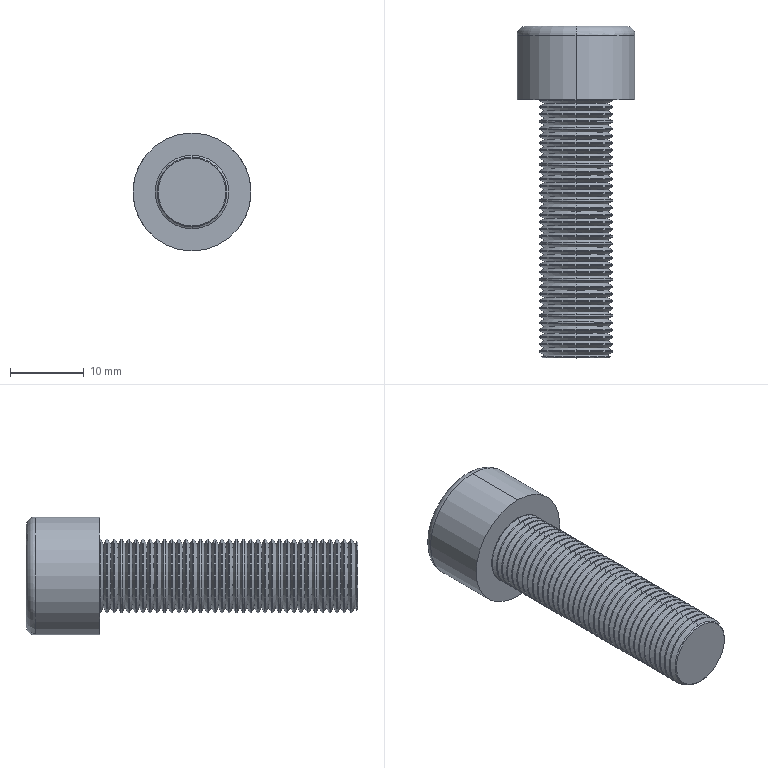Component | SolidWorks | HexagonSocketHeadCapScrew-M10X40-0510-3 | 1 solid | 239 faces | box 16 x 45 x 16 mm | volume 4119 mm3 | cone 148 | cylinder 74 | plane 15 | torus 2 | commonest cylinder face diameters 10 x72 16 x2
build123d program:
from build123d import *

# Parameters (mm, degrees)
SKETCH1_R           = 8
BASEHEAD_DEPTH      = 10
SKETCH2_R           = 5
BASEBODY_DEPTH      = 35
HEXAGONSOCKET_DEPTH = 5
TOPFILLET_R         = 1.25
CHAMFER1_SIZE       = 0.4
LPATTERN10_COUNT    = 36
LPATTERN10_PITCH    = 0.9744


with BuildPart() as part:
    # Sketch1 → BaseHead (new body)
    with BuildSketch(Plane(origin=(0, 0, 0), x_dir=(0, 0, -1), z_dir=(1, 0, 0))):
        Circle(SKETCH1_R)
    extrude(amount=BASEHEAD_DEPTH)

    # Sketch2 → BaseBody (add)
    with BuildSketch(Plane(origin=(10, 0, 0), x_dir=(0, 0, -1), z_dir=(1, 0, 0))):
        Circle(SKETCH2_R)
    extrude(amount=BASEBODY_DEPTH)

    # Sketch3 → HexagonSocket (cut)
    with BuildSketch(Plane(origin=(0, 0, 0), x_dir=(0, 0, -1), z_dir=(1, 0, 0))):
        Polygon((4.619, 0), (2.309, 4), (-2.309, 4), (-4.619, 0), (-2.309, -4), (2.309, -4), align=None)
    extrude(amount=HEXAGONSOCKET_DEPTH, mode=Mode.SUBTRACT)

    # Sketch4 → Cut-Revolve1 (revolve, cut)
    with BuildSketch(Plane(origin=(-4.196, 0.75, 0), x_dir=(-1, 0, 0), z_dir=(0, 0, 1)), mode=Mode.PRIVATE) as cut_revolve1_sk:
        Polygon((-9.196, 4.75), (-11.506, 0.75), (-9.196, 0.75), align=None)
    revolve(cut_revolve1_sk.sketch.rotate(Axis((0.839, 0, 0), (-1, 0, 0)), 90), axis=Axis((0.839, 0, 0), (-1, 0, 0)), mode=Mode.SUBTRACT)

    # TopFillet
    topfillet_edges = [part.edges().sort_by_distance(p)[0] for p in [
        (0, 0, 8),
    ]]
    fillet(topfillet_edges, radius=TOPFILLET_R)

    # Chamfer1
    chamfer1_edges = [part.edges().sort_by_distance(p)[0] for p in [
        (45, 0, 5),
    ]]
    chamfer(chamfer1_edges, length=CHAMFER1_SIZE)

    # Sketch5 → Cut-Revolve10 (revolve, cut)
    with BuildSketch(Plane.XY, mode=Mode.PRIVATE) as cut_revolve10_sk:
        Polygon((44.6, 4.297), (45.006, 5), (45.006, 5.812), (44.194, 5.812), (44.194, 5), align=None)
    cut_revolve10 = revolve(cut_revolve10_sk.sketch.rotate(Axis((0, 0, 0), (1, 0, 0)), 90), axis=Axis((0, 0, 0), (1, 0, 0)), mode=Mode.SUBTRACT)

    # LPattern10: Cut-Revolve10 ×36
    with Locations(*[(-i * LPATTERN10_PITCH, 0, 0) for i in range(1, LPATTERN10_COUNT)]):
        add(cut_revolve10, mode=Mode.SUBTRACT)


solid = part.part

# Placed as in the assembly
solid = solid.moved(Location((-857.7, 60.391, 3572.5), (0, 0, -90)))